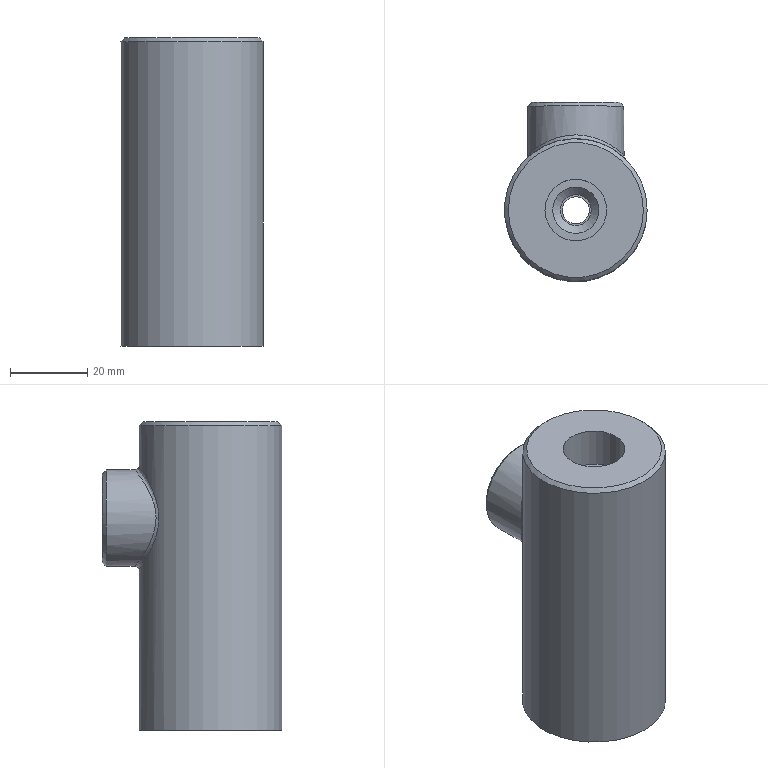Component | NX | VALVE_BODY | 1 solid | 21 faces | volume 63801 mm3 | cylinder 8 | cone 6 | plane 6 | spline 1 | commonest cylinder face diameters 7 x1 10.3 x1 37 x1 25 x1 20 x1 22.5 x1 16 x1 12 x1